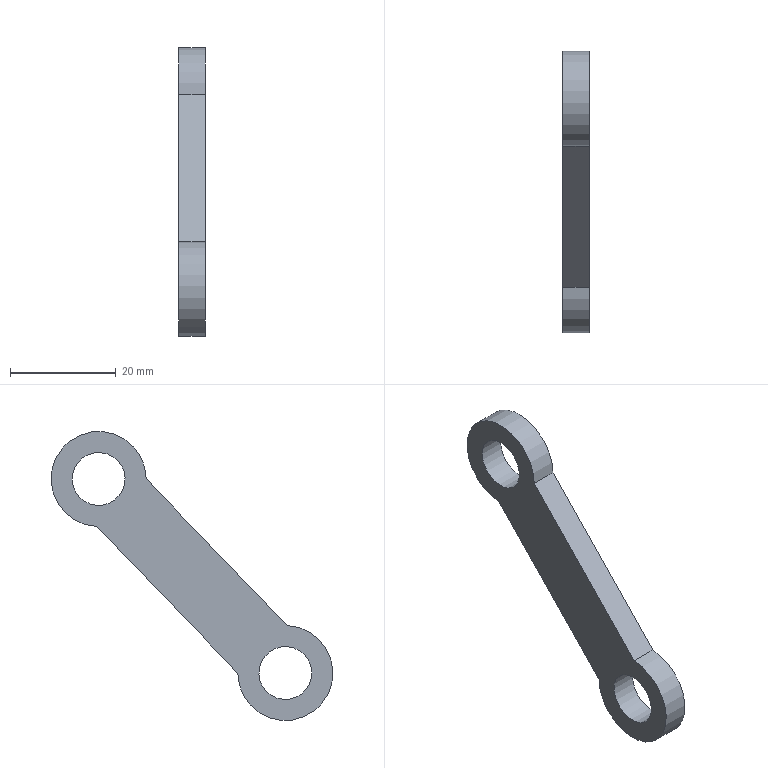Component | NX | CONNECTING_ROD | 1 solid | 8 faces | box 5 x 53.36 x 54.76 mm | volume 4016 mm3 | plane 4 | cylinder 4 | commonest cylinder face diameters 18 x2 10 x2
STEP:
#1=CARTESIAN_POINT('',(0.,0.,0.));
#2=DIRECTION('',(0.,0.,1.));
#3=DIRECTION('',(1.,0.,0.));
#4=AXIS2_PLACEMENT_3D('',#1,#2,#3);
#5=CARTESIAN_POINT('',(13.707,26.355,-109.336));
#6=VERTEX_POINT('',#5);
#7=CARTESIAN_POINT('',(13.707,-0.3692,-137.119));
#8=VERTEX_POINT('',#7);
#9=CARTESIAN_POINT('',(13.707,26.355,-109.336));
#10=DIRECTION('',(0.,-0.6932,-0.7207));
#11=VECTOR('',#10,1.);
#12=LINE('',#9,#11);
#13=CARTESIAN_POINT('',(18.707,26.355,-109.336));
#14=DIRECTION('',(0.,0.7207,-0.6932));
#15=DIRECTION('',(0.,0.6932,0.7207));
#16=AXIS2_PLACEMENT_3D('',#13,#14,#15);
#17=PLANE('',#16);
#18=CARTESIAN_POINT('',(0.,-5.));
#19=DIRECTION('',(-1.,0.));
#20=VECTOR('',#19,1.);
#21=LINE('',#18,#20);
#22=(GEOMETRIC_REPRESENTATION_CONTEXT(2)PARAMETRIC_REPRESENTATION_CONTEXT()REPRESENTATION_CONTEXT('',''));
#23=DEFINITIONAL_REPRESENTATION('',(#21),#22);
#24=PCURVE('',#17,#23);
#25=CARTESIAN_POINT('',(13.707,0.,-146.111));
#26=DIRECTION('',(1.,0.,0.));
#27=DIRECTION('',(0.,0.7207,-0.6932));
#28=AXIS2_PLACEMENT_3D('',#25,#26,#27);
#29=PLANE('',#28);
#30=CARTESIAN_POINT('',(-6.5,44.775));
#31=DIRECTION('',(0.,-1.));
#32=VECTOR('',#31,1.);
#33=LINE('',#30,#32);
#34=(GEOMETRIC_REPRESENTATION_CONTEXT(2)PARAMETRIC_REPRESENTATION_CONTEXT()REPRESENTATION_CONTEXT('',''));
#35=DEFINITIONAL_REPRESENTATION('',(#33),#34);
#36=PCURVE('',#29,#35);
#37=SURFACE_CURVE('',#12,(#24,#36),.PCURVE_S1.);
#38=EDGE_CURVE('',#6,#8,#37,.T.);
#39=ORIENTED_EDGE('',*,*,#38,.T.);
#40=CARTESIAN_POINT('',(18.707,-0.3692,-137.119));
#41=VERTEX_POINT('',#40);
#42=CARTESIAN_POINT('',(18.707,-0.3692,-137.119));
#43=DIRECTION('',(-1.,0.,0.));
#44=VECTOR('',#43,1.);
#45=LINE('',#42,#44);
#46=CARTESIAN_POINT('',(-38.55,0.));
#47=DIRECTION('',(0.,-1.));
#48=VECTOR('',#47,1.);
#49=LINE('',#46,#48);
#50=(GEOMETRIC_REPRESENTATION_CONTEXT(2)PARAMETRIC_REPRESENTATION_CONTEXT()REPRESENTATION_CONTEXT('',''));
#51=DEFINITIONAL_REPRESENTATION('',(#49),#50);
#52=PCURVE('',#17,#51);
#53=CARTESIAN_POINT('',(18.707,0.,-146.111));
#54=DIRECTION('',(-1.,0.,0.));
#55=DIRECTION('',(0.,-0.7207,0.6932));
#56=AXIS2_PLACEMENT_3D('',#53,#54,#55);
#57=CYLINDRICAL_SURFACE('',#56,9.);
#58=CARTESIAN_POINT('',(7.047,0.));
#59=DIRECTION('',(0.,1.));
#60=VECTOR('',#59,1.);
#61=LINE('',#58,#60);
#62=(GEOMETRIC_REPRESENTATION_CONTEXT(2)PARAMETRIC_REPRESENTATION_CONTEXT()REPRESENTATION_CONTEXT('',''));
#63=DEFINITIONAL_REPRESENTATION('',(#61),#62);
#64=PCURVE('',#57,#63);
#65=SURFACE_CURVE('',#45,(#52,#64),.PCURVE_S1.);
#66=EDGE_CURVE('',#41,#8,#65,.T.);
#67=ORIENTED_EDGE('',*,*,#66,.F.);
#68=CARTESIAN_POINT('',(18.707,26.355,-109.336));
#69=VERTEX_POINT('',#68);
#70=CARTESIAN_POINT('',(18.707,26.355,-109.336));
#71=DIRECTION('',(0.,-0.6932,-0.7207));
#72=VECTOR('',#71,1.);
#73=LINE('',#70,#72);
#74=CARTESIAN_POINT('',(0.,0.));
#75=DIRECTION('',(-1.,0.));
#76=VECTOR('',#75,1.);
#77=LINE('',#74,#76);
#78=(GEOMETRIC_REPRESENTATION_CONTEXT(2)PARAMETRIC_REPRESENTATION_CONTEXT()REPRESENTATION_CONTEXT('',''));
#79=DEFINITIONAL_REPRESENTATION('',(#77),#78);
#80=PCURVE('',#17,#79);
#81=CARTESIAN_POINT('',(18.707,0.,-146.111));
#82=DIRECTION('',(1.,0.,0.));
#83=DIRECTION('',(0.,0.7207,-0.6932));
#84=AXIS2_PLACEMENT_3D('',#81,#82,#83);
#85=PLANE('',#84);
#86=CARTESIAN_POINT('',(-6.5,44.775));
#87=DIRECTION('',(0.,-1.));
#88=VECTOR('',#87,1.);
#89=LINE('',#86,#88);
#90=(GEOMETRIC_REPRESENTATION_CONTEXT(2)PARAMETRIC_REPRESENTATION_CONTEXT()REPRESENTATION_CONTEXT('',''));
#91=DEFINITIONAL_REPRESENTATION('',(#89),#90);
#92=PCURVE('',#85,#91);
#93=SURFACE_CURVE('',#73,(#80,#92),.PCURVE_S1.);
#94=EDGE_CURVE('',#69,#41,#93,.T.);
#95=ORIENTED_EDGE('',*,*,#94,.F.);
#96=CARTESIAN_POINT('',(18.707,26.355,-109.336));
#97=DIRECTION('',(-1.,0.,0.));
#98=VECTOR('',#97,1.);
#99=LINE('',#96,#98);
#100=CARTESIAN_POINT('',(0.,0.));
#101=DIRECTION('',(0.,-1.));
#102=VECTOR('',#101,1.);
#103=LINE('',#100,#102);
#104=(GEOMETRIC_REPRESENTATION_CONTEXT(2)PARAMETRIC_REPRESENTATION_CONTEXT()REPRESENTATION_CONTEXT('',''));
#105=DEFINITIONAL_REPRESENTATION('',(#103),#104);
#106=PCURVE('',#17,#105);
#107=CARTESIAN_POINT('',(18.707,35.355,-109.355));
#108=DIRECTION('',(-1.,0.,0.));
#109=DIRECTION('',(0.,-0.7207,0.6932));
#110=AXIS2_PLACEMENT_3D('',#107,#108,#109);
#111=CYLINDRICAL_SURFACE('',#110,9.);
#112=CARTESIAN_POINT('',(-0.7638,0.));
#113=DIRECTION('',(0.,1.));
#114=VECTOR('',#113,1.);
#115=LINE('',#112,#114);
#116=(GEOMETRIC_REPRESENTATION_CONTEXT(2)PARAMETRIC_REPRESENTATION_CONTEXT()REPRESENTATION_CONTEXT('',''));
#117=DEFINITIONAL_REPRESENTATION('',(#115),#116);
#118=PCURVE('',#111,#117);
#119=SURFACE_CURVE('',#99,(#106,#118),.PCURVE_S1.);
#120=EDGE_CURVE('',#69,#6,#119,.T.);
#121=ORIENTED_EDGE('',*,*,#120,.T.);
#122=EDGE_LOOP('',(#39,#67,#95,#121));
#123=FACE_BOUND('',#122,.T.);
#124=ADVANCED_FACE('',(#123),#17,.F.);
#125=CARTESIAN_POINT('',(13.707,9.,-146.131));
#126=VERTEX_POINT('',#125);
#127=CARTESIAN_POINT('',(13.707,0.,-146.111));
#128=DIRECTION('',(1.,0.,0.));
#129=DIRECTION('',(0.,0.7207,-0.6932));
#130=AXIS2_PLACEMENT_3D('',#127,#128,#129);
#131=CIRCLE('',#130,9.);
#132=CARTESIAN_POINT('',(9.425,5.));
#133=DIRECTION('',(-1.,0.));
#134=VECTOR('',#133,1.);
#135=LINE('',#132,#134);
#136=(GEOMETRIC_REPRESENTATION_CONTEXT(2)PARAMETRIC_REPRESENTATION_CONTEXT()REPRESENTATION_CONTEXT('',''));
#137=DEFINITIONAL_REPRESENTATION('',(#135),#136);
#138=PCURVE('',#57,#137);
#139=CARTESIAN_POINT('',(0.,0.));
#140=DIRECTION('',(1.,-0.));
#141=AXIS2_PLACEMENT_2D('',#139,#140);
#142=CIRCLE('',#141,9.);
#143=(GEOMETRIC_REPRESENTATION_CONTEXT(2)PARAMETRIC_REPRESENTATION_CONTEXT()REPRESENTATION_CONTEXT('',''));
#144=DEFINITIONAL_REPRESENTATION('',(#142),#143);
#145=PCURVE('',#29,#144);
#146=SURFACE_CURVE('',#131,(#138,#145),.PCURVE_S1.);
#147=EDGE_CURVE('',#8,#126,#146,.T.);
#148=ORIENTED_EDGE('',*,*,#147,.T.);
#149=CARTESIAN_POINT('',(18.707,9.,-146.131));
#150=VERTEX_POINT('',#149);
#151=CARTESIAN_POINT('',(18.707,9.,-146.131));
#152=DIRECTION('',(-1.,0.,0.));
#153=VECTOR('',#152,1.);
#154=LINE('',#151,#153);
#155=CARTESIAN_POINT('',(2.378,0.));
#156=DIRECTION('',(0.,1.));
#157=VECTOR('',#156,1.);
#158=LINE('',#155,#157);
#159=(GEOMETRIC_REPRESENTATION_CONTEXT(2)PARAMETRIC_REPRESENTATION_CONTEXT()REPRESENTATION_CONTEXT('',''));
#160=DEFINITIONAL_REPRESENTATION('',(#158),#159);
#161=PCURVE('',#57,#160);
#162=CARTESIAN_POINT('',(18.707,9.,-146.131));
#163=DIRECTION('',(0.,-0.7207,0.6932));
#164=DIRECTION('',(0.,-0.6932,-0.7207));
#165=AXIS2_PLACEMENT_3D('',#162,#163,#164);
#166=PLANE('',#165);
#167=CARTESIAN_POINT('',(-0.,0.));
#168=DIRECTION('',(0.,-1.));
#169=VECTOR('',#168,1.);
#170=LINE('',#167,#169);
#171=(GEOMETRIC_REPRESENTATION_CONTEXT(2)PARAMETRIC_REPRESENTATION_CONTEXT()REPRESENTATION_CONTEXT('',''));
#172=DEFINITIONAL_REPRESENTATION('',(#170),#171);
#173=PCURVE('',#166,#172);
#174=SURFACE_CURVE('',#154,(#161,#173),.PCURVE_S1.);
#175=EDGE_CURVE('',#150,#126,#174,.T.);
#176=ORIENTED_EDGE('',*,*,#175,.F.);
#177=CARTESIAN_POINT('',(18.707,0.,-146.111));
#178=DIRECTION('',(1.,0.,0.));
#179=DIRECTION('',(0.,0.7207,-0.6932));
#180=AXIS2_PLACEMENT_3D('',#177,#178,#179);
#181=CIRCLE('',#180,9.);
#182=CARTESIAN_POINT('',(9.425,0.));
#183=DIRECTION('',(-1.,0.));
#184=VECTOR('',#183,1.);
#185=LINE('',#182,#184);
#186=(GEOMETRIC_REPRESENTATION_CONTEXT(2)PARAMETRIC_REPRESENTATION_CONTEXT()REPRESENTATION_CONTEXT('',''));
#187=DEFINITIONAL_REPRESENTATION('',(#185),#186);
#188=PCURVE('',#57,#187);
#189=CARTESIAN_POINT('',(0.,0.));
#190=DIRECTION('',(1.,-0.));
#191=AXIS2_PLACEMENT_2D('',#189,#190);
#192=CIRCLE('',#191,9.);
#193=(GEOMETRIC_REPRESENTATION_CONTEXT(2)PARAMETRIC_REPRESENTATION_CONTEXT()REPRESENTATION_CONTEXT('',''));
#194=DEFINITIONAL_REPRESENTATION('',(#192),#193);
#195=PCURVE('',#85,#194);
#196=SURFACE_CURVE('',#181,(#188,#195),.PCURVE_S1.);
#197=EDGE_CURVE('',#41,#150,#196,.T.);
#198=ORIENTED_EDGE('',*,*,#197,.F.);
#199=ORIENTED_EDGE('',*,*,#66,.T.);
#200=EDGE_LOOP('',(#148,#176,#198,#199));
#201=FACE_BOUND('',#200,.T.);
#202=ADVANCED_FACE('',(#201),#57,.T.);
#203=CARTESIAN_POINT('',(13.707,35.725,-118.348));
#204=VERTEX_POINT('',#203);
#205=CARTESIAN_POINT('',(13.707,9.,-146.131));
#206=DIRECTION('',(0.,0.6932,0.7207));
#207=VECTOR('',#206,1.);
#208=LINE('',#205,#207);
#209=CARTESIAN_POINT('',(0.,-5.));
#210=DIRECTION('',(-1.,0.));
#211=VECTOR('',#210,1.);
#212=LINE('',#209,#211);
#213=(GEOMETRIC_REPRESENTATION_CONTEXT(2)PARAMETRIC_REPRESENTATION_CONTEXT()REPRESENTATION_CONTEXT('',''));
#214=DEFINITIONAL_REPRESENTATION('',(#212),#213);
#215=PCURVE('',#166,#214);
#216=CARTESIAN_POINT('',(6.5,6.225));
#217=DIRECTION('',(0.,1.));
#218=VECTOR('',#217,1.);
#219=LINE('',#216,#218);
#220=(GEOMETRIC_REPRESENTATION_CONTEXT(2)PARAMETRIC_REPRESENTATION_CONTEXT()REPRESENTATION_CONTEXT('',''));
#221=DEFINITIONAL_REPRESENTATION('',(#219),#220);
#222=PCURVE('',#29,#221);
#223=SURFACE_CURVE('',#208,(#215,#222),.PCURVE_S1.);
#224=EDGE_CURVE('',#126,#204,#223,.T.);
#225=ORIENTED_EDGE('',*,*,#224,.T.);
#226=CARTESIAN_POINT('',(18.707,35.725,-118.348));
#227=VERTEX_POINT('',#226);
#228=CARTESIAN_POINT('',(18.707,35.725,-118.348));
#229=DIRECTION('',(-1.,0.,0.));
#230=VECTOR('',#229,1.);
#231=LINE('',#228,#230);
#232=CARTESIAN_POINT('',(-38.55,0.));
#233=DIRECTION('',(0.,-1.));
#234=VECTOR('',#233,1.);
#235=LINE('',#232,#234);
#236=(GEOMETRIC_REPRESENTATION_CONTEXT(2)PARAMETRIC_REPRESENTATION_CONTEXT()REPRESENTATION_CONTEXT('',''));
#237=DEFINITIONAL_REPRESENTATION('',(#235),#236);
#238=PCURVE('',#166,#237);
#239=CARTESIAN_POINT('',(3.905,0.));
#240=DIRECTION('',(0.,1.));
#241=VECTOR('',#240,1.);
#242=LINE('',#239,#241);
#243=(GEOMETRIC_REPRESENTATION_CONTEXT(2)PARAMETRIC_REPRESENTATION_CONTEXT()REPRESENTATION_CONTEXT('',''));
#244=DEFINITIONAL_REPRESENTATION('',(#242),#243);
#245=PCURVE('',#111,#244);
#246=SURFACE_CURVE('',#231,(#238,#245),.PCURVE_S1.);
#247=EDGE_CURVE('',#227,#204,#246,.T.);
#248=ORIENTED_EDGE('',*,*,#247,.F.);
#249=CARTESIAN_POINT('',(18.707,9.,-146.131));
#250=DIRECTION('',(0.,0.6932,0.7207));
#251=VECTOR('',#250,1.);
#252=LINE('',#249,#251);
#253=CARTESIAN_POINT('',(0.,0.));
#254=DIRECTION('',(-1.,0.));
#255=VECTOR('',#254,1.);
#256=LINE('',#253,#255);
#257=(GEOMETRIC_REPRESENTATION_CONTEXT(2)PARAMETRIC_REPRESENTATION_CONTEXT()REPRESENTATION_CONTEXT('',''));
#258=DEFINITIONAL_REPRESENTATION('',(#256),#257);
#259=PCURVE('',#166,#258);
#260=CARTESIAN_POINT('',(6.5,6.225));
#261=DIRECTION('',(0.,1.));
#262=VECTOR('',#261,1.);
#263=LINE('',#260,#262);
#264=(GEOMETRIC_REPRESENTATION_CONTEXT(2)PARAMETRIC_REPRESENTATION_CONTEXT()REPRESENTATION_CONTEXT('',''));
#265=DEFINITIONAL_REPRESENTATION('',(#263),#264);
#266=PCURVE('',#85,#265);
#267=SURFACE_CURVE('',#252,(#259,#266),.PCURVE_S1.);
#268=EDGE_CURVE('',#150,#227,#267,.T.);
#269=ORIENTED_EDGE('',*,*,#268,.F.);
#270=ORIENTED_EDGE('',*,*,#175,.T.);
#271=EDGE_LOOP('',(#225,#248,#269,#270));
#272=FACE_BOUND('',#271,.T.);
#273=ADVANCED_FACE('',(#272),#166,.F.);
#274=CARTESIAN_POINT('',(18.707,3.604,-149.578));
#275=VERTEX_POINT('',#274);
#276=CARTESIAN_POINT('',(18.707,0.,-146.111));
#277=DIRECTION('',(-1.,0.,0.));
#278=DIRECTION('',(0.,0.7207,-0.6932));
#279=AXIS2_PLACEMENT_3D('',#276,#277,#278);
#280=CIRCLE('',#279,5.);
#281=CARTESIAN_POINT('',(18.707,0.,-146.111));
#282=DIRECTION('',(-1.,0.,0.));
#283=DIRECTION('',(0.,-0.7207,0.6932));
#284=AXIS2_PLACEMENT_3D('',#281,#282,#283);
#285=CYLINDRICAL_SURFACE('',#284,5.);
#286=CARTESIAN_POINT('',(3.142,0.));
#287=DIRECTION('',(1.,0.));
#288=VECTOR('',#287,1.);
#289=LINE('',#286,#288);
#290=(GEOMETRIC_REPRESENTATION_CONTEXT(2)PARAMETRIC_REPRESENTATION_CONTEXT()REPRESENTATION_CONTEXT('',''));
#291=DEFINITIONAL_REPRESENTATION('',(#289),#290);
#292=PCURVE('',#285,#291);
#293=CARTESIAN_POINT('',(5.,-0.));
#294=CARTESIAN_POINT('',(5.,-8.66));
#295=CARTESIAN_POINT('',(-2.5,-4.33));
#296=CARTESIAN_POINT('',(-10.,0.));
#297=CARTESIAN_POINT('',(-2.5,4.33));
#298=CARTESIAN_POINT('',(5.,8.66));
#299=CARTESIAN_POINT('',(5.,-0.));
#300=(BOUNDED_CURVE()B_SPLINE_CURVE(2,(#293,#294,#295,#296,#297,#298,#299),.UNSPECIFIED.,.T.,.F.)B_SPLINE_CURVE_WITH_KNOTS((1,2,2,2,2,1),(-2.094,0.,2.094,4.189,6.283,8.378),.UNSPECIFIED.)CURVE()GEOMETRIC_REPRESENTATION_ITEM()RATIONAL_B_SPLINE_CURVE((1.,0.5,1.,0.5,1.,0.5,1.))REPRESENTATION_ITEM(''));
#301=(GEOMETRIC_REPRESENTATION_CONTEXT(2)PARAMETRIC_REPRESENTATION_CONTEXT()REPRESENTATION_CONTEXT('',''));
#302=DEFINITIONAL_REPRESENTATION('',(#300),#301);
#303=PCURVE('',#85,#302);
#304=SURFACE_CURVE('',#280,(#292,#303),.PCURVE_S1.);
#305=EDGE_CURVE('',#275,#275,#304,.T.);
#306=ORIENTED_EDGE('',*,*,#305,.T.);
#307=CARTESIAN_POINT('',(13.707,3.604,-149.578));
#308=VERTEX_POINT('',#307);
#309=CARTESIAN_POINT('',(18.707,3.604,-149.578));
#310=CARTESIAN_POINT('',(13.707,3.604,-149.578));
#311=B_SPLINE_CURVE_WITH_KNOTS('',1,(#309,#310),.UNSPECIFIED.,.F.,.F.,(2,2),(0.,5.),.PIECEWISE_BEZIER_KNOTS.);
#312=CARTESIAN_POINT('',(9.425,0.));
#313=DIRECTION('',(0.,1.));
#314=VECTOR('',#313,1.);
#315=LINE('',#312,#314);
#316=(GEOMETRIC_REPRESENTATION_CONTEXT(2)PARAMETRIC_REPRESENTATION_CONTEXT()REPRESENTATION_CONTEXT('',''));
#317=DEFINITIONAL_REPRESENTATION('',(#315),#316);
#318=PCURVE('',#285,#317);
#319=CARTESIAN_POINT('',(3.142,0.));
#320=DIRECTION('',(0.,1.));
#321=VECTOR('',#320,1.);
#322=LINE('',#319,#321);
#323=(GEOMETRIC_REPRESENTATION_CONTEXT(2)PARAMETRIC_REPRESENTATION_CONTEXT()REPRESENTATION_CONTEXT('',''));
#324=DEFINITIONAL_REPRESENTATION('',(#322),#323);
#325=PCURVE('',#285,#324);
#326=SEAM_CURVE('',#311,(#318,#325),.PCURVE_S1.);
#327=EDGE_CURVE('',#275,#308,#326,.T.);
#328=ORIENTED_EDGE('',*,*,#327,.T.);
#329=CARTESIAN_POINT('',(13.707,0.,-146.111));
#330=DIRECTION('',(-1.,0.,0.));
#331=DIRECTION('',(0.,0.7207,-0.6932));
#332=AXIS2_PLACEMENT_3D('',#329,#330,#331);
#333=CIRCLE('',#332,5.);
#334=CARTESIAN_POINT('',(3.142,5.));
#335=DIRECTION('',(1.,0.));
#336=VECTOR('',#335,1.);
#337=LINE('',#334,#336);
#338=(GEOMETRIC_REPRESENTATION_CONTEXT(2)PARAMETRIC_REPRESENTATION_CONTEXT()REPRESENTATION_CONTEXT('',''));
#339=DEFINITIONAL_REPRESENTATION('',(#337),#338);
#340=PCURVE('',#285,#339);
#341=CARTESIAN_POINT('',(5.,-0.));
#342=CARTESIAN_POINT('',(5.,-8.66));
#343=CARTESIAN_POINT('',(-2.5,-4.33));
#344=CARTESIAN_POINT('',(-10.,0.));
#345=CARTESIAN_POINT('',(-2.5,4.33));
#346=CARTESIAN_POINT('',(5.,8.66));
#347=CARTESIAN_POINT('',(5.,-0.));
#348=(BOUNDED_CURVE()B_SPLINE_CURVE(2,(#341,#342,#343,#344,#345,#346,#347),.UNSPECIFIED.,.T.,.F.)B_SPLINE_CURVE_WITH_KNOTS((1,2,2,2,2,1),(-2.094,0.,2.094,4.189,6.283,8.378),.UNSPECIFIED.)CURVE()GEOMETRIC_REPRESENTATION_ITEM()RATIONAL_B_SPLINE_CURVE((1.,0.5,1.,0.5,1.,0.5,1.))REPRESENTATION_ITEM(''));
#349=(GEOMETRIC_REPRESENTATION_CONTEXT(2)PARAMETRIC_REPRESENTATION_CONTEXT()REPRESENTATION_CONTEXT('',''));
#350=DEFINITIONAL_REPRESENTATION('',(#348),#349);
#351=PCURVE('',#29,#350);
#352=SURFACE_CURVE('',#333,(#340,#351),.PCURVE_S1.);
#353=EDGE_CURVE('',#308,#308,#352,.T.);
#354=ORIENTED_EDGE('',*,*,#353,.F.);
#355=ORIENTED_EDGE('',*,*,#327,.F.);
#356=EDGE_LOOP('',(#306,#328,#354,#355));
#357=FACE_BOUND('',#356,.F.);
#358=ADVANCED_FACE('',(#357),#285,.F.);
#359=CARTESIAN_POINT('',(13.707,35.355,-109.355));
#360=DIRECTION('',(1.,0.,0.));
#361=DIRECTION('',(0.,0.7207,-0.6932));
#362=AXIS2_PLACEMENT_3D('',#359,#360,#361);
#363=CIRCLE('',#362,9.);
#364=CARTESIAN_POINT('',(9.425,5.));
#365=DIRECTION('',(-1.,0.));
#366=VECTOR('',#365,1.);
#367=LINE('',#364,#366);
#368=(GEOMETRIC_REPRESENTATION_CONTEXT(2)PARAMETRIC_REPRESENTATION_CONTEXT()REPRESENTATION_CONTEXT('',''));
#369=DEFINITIONAL_REPRESENTATION('',(#367),#368);
#370=PCURVE('',#111,#369);
#371=CARTESIAN_POINT('',(0.,51.));
#372=DIRECTION('',(1.,-0.));
#373=AXIS2_PLACEMENT_2D('',#371,#372);
#374=CIRCLE('',#373,9.);
#375=(GEOMETRIC_REPRESENTATION_CONTEXT(2)PARAMETRIC_REPRESENTATION_CONTEXT()REPRESENTATION_CONTEXT('',''));
#376=DEFINITIONAL_REPRESENTATION('',(#374),#375);
#377=PCURVE('',#29,#376);
#378=SURFACE_CURVE('',#363,(#370,#377),.PCURVE_S1.);
#379=EDGE_CURVE('',#204,#6,#378,.T.);
#380=ORIENTED_EDGE('',*,*,#379,.T.);
#381=ORIENTED_EDGE('',*,*,#120,.F.);
#382=CARTESIAN_POINT('',(18.707,35.355,-109.355));
#383=DIRECTION('',(1.,0.,0.));
#384=DIRECTION('',(0.,0.7207,-0.6932));
#385=AXIS2_PLACEMENT_3D('',#382,#383,#384);
#386=CIRCLE('',#385,9.);
#387=CARTESIAN_POINT('',(9.425,0.));
#388=DIRECTION('',(-1.,0.));
#389=VECTOR('',#388,1.);
#390=LINE('',#387,#389);
#391=(GEOMETRIC_REPRESENTATION_CONTEXT(2)PARAMETRIC_REPRESENTATION_CONTEXT()REPRESENTATION_CONTEXT('',''));
#392=DEFINITIONAL_REPRESENTATION('',(#390),#391);
#393=PCURVE('',#111,#392);
#394=CARTESIAN_POINT('',(0.,51.));
#395=DIRECTION('',(1.,-0.));
#396=AXIS2_PLACEMENT_2D('',#394,#395);
#397=CIRCLE('',#396,9.);
#398=(GEOMETRIC_REPRESENTATION_CONTEXT(2)PARAMETRIC_REPRESENTATION_CONTEXT()REPRESENTATION_CONTEXT('',''));
#399=DEFINITIONAL_REPRESENTATION('',(#397),#398);
#400=PCURVE('',#85,#399);
#401=SURFACE_CURVE('',#386,(#393,#400),.PCURVE_S1.);
#402=EDGE_CURVE('',#227,#69,#401,.T.);
#403=ORIENTED_EDGE('',*,*,#402,.F.);
#404=ORIENTED_EDGE('',*,*,#247,.T.);
#405=EDGE_LOOP('',(#380,#381,#403,#404));
#406=FACE_BOUND('',#405,.T.);
#407=ADVANCED_FACE('',(#406),#111,.T.);
#408=CARTESIAN_POINT('',(18.707,38.959,-112.822));
#409=VERTEX_POINT('',#408);
#410=CARTESIAN_POINT('',(18.707,35.355,-109.355));
#411=DIRECTION('',(1.,0.,0.));
#412=DIRECTION('',(0.,0.7207,-0.6932));
#413=AXIS2_PLACEMENT_3D('',#410,#411,#412);
#414=CIRCLE('',#413,5.);
#415=CARTESIAN_POINT('',(18.707,35.355,-109.355));
#416=DIRECTION('',(-1.,0.,0.));
#417=DIRECTION('',(0.,-0.7207,0.6932));
#418=AXIS2_PLACEMENT_3D('',#415,#416,#417);
#419=CYLINDRICAL_SURFACE('',#418,5.);
#420=CARTESIAN_POINT('',(9.425,0.));
#421=DIRECTION('',(-1.,0.));
#422=VECTOR('',#421,1.);
#423=LINE('',#420,#422);
#424=(GEOMETRIC_REPRESENTATION_CONTEXT(2)PARAMETRIC_REPRESENTATION_CONTEXT()REPRESENTATION_CONTEXT('',''));
#425=DEFINITIONAL_REPRESENTATION('',(#423),#424);
#426=PCURVE('',#419,#425);
#427=CARTESIAN_POINT('',(0.,51.));
#428=DIRECTION('',(1.,-0.));
#429=AXIS2_PLACEMENT_2D('',#427,#428);
#430=CIRCLE('',#429,5.);
#431=(GEOMETRIC_REPRESENTATION_CONTEXT(2)PARAMETRIC_REPRESENTATION_CONTEXT()REPRESENTATION_CONTEXT('',''));
#432=DEFINITIONAL_REPRESENTATION('',(#430),#431);
#433=PCURVE('',#85,#432);
#434=SURFACE_CURVE('',#414,(#426,#433),.PCURVE_S1.);
#435=EDGE_CURVE('',#409,#409,#434,.T.);
#436=ORIENTED_EDGE('',*,*,#435,.F.);
#437=CARTESIAN_POINT('',(13.707,38.959,-112.822));
#438=VERTEX_POINT('',#437);
#439=CARTESIAN_POINT('',(18.707,38.959,-112.822));
#440=CARTESIAN_POINT('',(13.707,38.959,-112.822));
#441=B_SPLINE_CURVE_WITH_KNOTS('',1,(#439,#440),.UNSPECIFIED.,.F.,.F.,(2,2),(0.,5.),.PIECEWISE_BEZIER_KNOTS.);
#442=CARTESIAN_POINT('',(9.425,0.));
#443=DIRECTION('',(0.,1.));
#444=VECTOR('',#443,1.);
#445=LINE('',#442,#444);
#446=(GEOMETRIC_REPRESENTATION_CONTEXT(2)PARAMETRIC_REPRESENTATION_CONTEXT()REPRESENTATION_CONTEXT('',''));
#447=DEFINITIONAL_REPRESENTATION('',(#445),#446);
#448=PCURVE('',#419,#447);
#449=CARTESIAN_POINT('',(3.142,0.));
#450=DIRECTION('',(0.,1.));
#451=VECTOR('',#450,1.);
#452=LINE('',#449,#451);
#453=(GEOMETRIC_REPRESENTATION_CONTEXT(2)PARAMETRIC_REPRESENTATION_CONTEXT()REPRESENTATION_CONTEXT('',''));
#454=DEFINITIONAL_REPRESENTATION('',(#452),#453);
#455=PCURVE('',#419,#454);
#456=SEAM_CURVE('',#441,(#448,#455),.PCURVE_S1.);
#457=EDGE_CURVE('',#409,#438,#456,.T.);
#458=ORIENTED_EDGE('',*,*,#457,.T.);
#459=CARTESIAN_POINT('',(13.707,35.355,-109.355));
#460=DIRECTION('',(1.,0.,0.));
#461=DIRECTION('',(0.,0.7207,-0.6932));
#462=AXIS2_PLACEMENT_3D('',#459,#460,#461);
#463=CIRCLE('',#462,5.);
#464=CARTESIAN_POINT('',(9.425,5.));
#465=DIRECTION('',(-1.,0.));
#466=VECTOR('',#465,1.);
#467=LINE('',#464,#466);
#468=(GEOMETRIC_REPRESENTATION_CONTEXT(2)PARAMETRIC_REPRESENTATION_CONTEXT()REPRESENTATION_CONTEXT('',''));
#469=DEFINITIONAL_REPRESENTATION('',(#467),#468);
#470=PCURVE('',#419,#469);
#471=CARTESIAN_POINT('',(0.,51.));
#472=DIRECTION('',(1.,-0.));
#473=AXIS2_PLACEMENT_2D('',#471,#472);
#474=CIRCLE('',#473,5.);
#475=(GEOMETRIC_REPRESENTATION_CONTEXT(2)PARAMETRIC_REPRESENTATION_CONTEXT()REPRESENTATION_CONTEXT('',''));
#476=DEFINITIONAL_REPRESENTATION('',(#474),#475);
#477=PCURVE('',#29,#476);
#478=SURFACE_CURVE('',#463,(#470,#477),.PCURVE_S1.);
#479=EDGE_CURVE('',#438,#438,#478,.T.);
#480=ORIENTED_EDGE('',*,*,#479,.T.);
#481=ORIENTED_EDGE('',*,*,#457,.F.);
#482=EDGE_LOOP('',(#436,#458,#480,#481));
#483=FACE_BOUND('',#482,.F.);
#484=ADVANCED_FACE('',(#483),#419,.F.);
#485=ORIENTED_EDGE('',*,*,#94,.T.);
#486=ORIENTED_EDGE('',*,*,#197,.T.);
#487=ORIENTED_EDGE('',*,*,#268,.T.);
#488=ORIENTED_EDGE('',*,*,#402,.T.);
#489=EDGE_LOOP('',(#485,#486,#487,#488));
#490=FACE_BOUND('',#489,.T.);
#491=ORIENTED_EDGE('',*,*,#305,.T.);
#492=EDGE_LOOP('',(#491));
#493=FACE_BOUND('',#492,.T.);
#494=ORIENTED_EDGE('',*,*,#435,.F.);
#495=EDGE_LOOP('',(#494));
#496=FACE_BOUND('',#495,.T.);
#497=ADVANCED_FACE('',(#490,#493,#496),#85,.T.);
#498=ORIENTED_EDGE('',*,*,#38,.F.);
#499=ORIENTED_EDGE('',*,*,#379,.F.);
#500=ORIENTED_EDGE('',*,*,#224,.F.);
#501=ORIENTED_EDGE('',*,*,#147,.F.);
#502=EDGE_LOOP('',(#498,#499,#500,#501));
#503=FACE_BOUND('',#502,.T.);
#504=ORIENTED_EDGE('',*,*,#353,.F.);
#505=EDGE_LOOP('',(#504));
#506=FACE_BOUND('',#505,.T.);
#507=ORIENTED_EDGE('',*,*,#479,.T.);
#508=EDGE_LOOP('',(#507));
#509=FACE_BOUND('',#508,.T.);
#510=ADVANCED_FACE('',(#503,#506,#509),#29,.F.);
#511=CLOSED_SHELL('',(#124,#202,#273,#358,#407,#484,#497,#510));
#512=MANIFOLD_SOLID_BREP('',#511);
#513=(LENGTH_UNIT()NAMED_UNIT(*)SI_UNIT(.MILLI.,.METRE.));
#514=UNCERTAINTY_MEASURE_WITH_UNIT(LENGTH_MEASURE(0.000002),#513,'','');
#515=(NAMED_UNIT(*)PLANE_ANGLE_UNIT()SI_UNIT($,.RADIAN.));
#516=(NAMED_UNIT(*)SI_UNIT($,.STERADIAN.)SOLID_ANGLE_UNIT());
#517=(GEOMETRIC_REPRESENTATION_CONTEXT(3)GLOBAL_UNCERTAINTY_ASSIGNED_CONTEXT((#514))GLOBAL_UNIT_ASSIGNED_CONTEXT((#513,#515,#516))REPRESENTATION_CONTEXT('',''));
#518=ADVANCED_BREP_SHAPE_REPRESENTATION('',(#4,#512),#517);